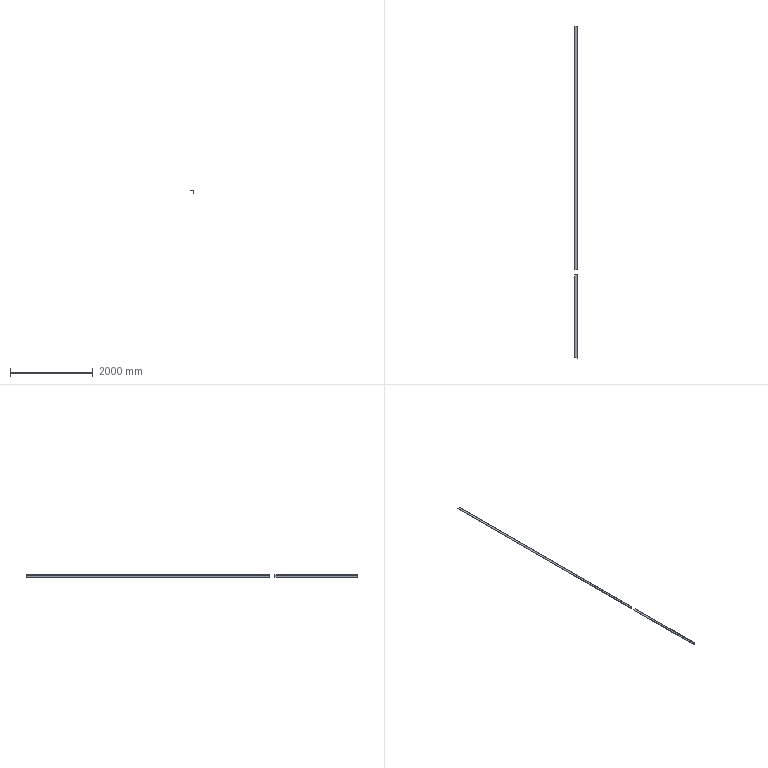Component | SolidWorks | 63#AngleIron-1 | 2 solids | 22 faces | box 63 x 8000 x 63 mm | volume 3919801 mm3 | plane 16 | cylinder 6 | commonest cylinder face diameters 2.667 x4 14 x2
STEP:
#1=CARTESIAN_POINT('',(81.493,-204.522,184.882));
#2=VERTEX_POINT('',#1);
#3=CARTESIAN_POINT('',(81.493,-283.262,184.882));
#4=VERTEX_POINT('',#3);
#5=CARTESIAN_POINT('',(81.493,31.699,184.882));
#6=DIRECTION('',(-0.,-1.,0.));
#7=VECTOR('',#6,39.37);
#8=LINE('',#5,#7);
#9=EDGE_CURVE('',#2,#4,#8,.T.);
#10=ORIENTED_EDGE('',*,*,#9,.F.);
#11=CARTESIAN_POINT('',(81.493,-204.522,187.362));
#12=VERTEX_POINT('',#11);
#13=CARTESIAN_POINT('',(81.493,-204.522,184.882));
#14=DIRECTION('',(0.,0.,1.));
#15=VECTOR('',#14,39.37);
#16=LINE('',#13,#15);
#17=EDGE_CURVE('',#2,#12,#16,.T.);
#18=ORIENTED_EDGE('',*,*,#17,.T.);
#19=CARTESIAN_POINT('',(81.493,-283.262,187.362));
#20=VERTEX_POINT('',#19);
#21=CARTESIAN_POINT('',(81.493,31.699,187.362));
#22=DIRECTION('',(-0.,-1.,0.));
#23=VECTOR('',#22,39.37);
#24=LINE('',#21,#23);
#25=EDGE_CURVE('',#12,#20,#24,.T.);
#26=ORIENTED_EDGE('',*,*,#25,.T.);
#27=CARTESIAN_POINT('',(81.493,-283.262,184.882));
#28=DIRECTION('',(-0.,-0.,-1.));
#29=VECTOR('',#28,39.37);
#30=LINE('',#27,#29);
#31=EDGE_CURVE('',#20,#4,#30,.T.);
#32=ORIENTED_EDGE('',*,*,#31,.T.);
#33=EDGE_LOOP('',(#10,#18,#26,#32));
#34=FACE_OUTER_BOUND('',#33,.T.);
#35=CARTESIAN_POINT('',(81.493,31.699,184.882));
#36=DIRECTION('',(-1.,0.,0.));
#37=DIRECTION('',(0.,1.,-0.));
#38=AXIS2_PLACEMENT_3D('',#35,#36,#37);
#39=PLANE('',#38);
#40=ADVANCED_FACE('',(#34),#39,.F.);
#41=CARTESIAN_POINT('',(81.388,-204.522,184.882));
#42=VERTEX_POINT('',#41);
#43=CARTESIAN_POINT('',(81.388,-283.262,184.882));
#44=VERTEX_POINT('',#43);
#45=CARTESIAN_POINT('',(81.388,31.699,184.882));
#46=DIRECTION('',(-0.,-1.,0.));
#47=VECTOR('',#46,39.37);
#48=LINE('',#45,#47);
#49=EDGE_CURVE('',#42,#44,#48,.T.);
#50=ORIENTED_EDGE('',*,*,#49,.F.);
#51=CARTESIAN_POINT('',(81.493,-204.522,184.882));
#52=DIRECTION('',(1.,0.,-0.));
#53=VECTOR('',#52,39.37);
#54=LINE('',#51,#53);
#55=EDGE_CURVE('',#42,#2,#54,.T.);
#56=ORIENTED_EDGE('',*,*,#55,.T.);
#57=ORIENTED_EDGE('',*,*,#9,.T.);
#58=CARTESIAN_POINT('',(81.493,-283.262,184.882));
#59=DIRECTION('',(-1.,0.,0.));
#60=VECTOR('',#59,39.37);
#61=LINE('',#58,#60);
#62=EDGE_CURVE('',#4,#44,#61,.T.);
#63=ORIENTED_EDGE('',*,*,#62,.T.);
#64=EDGE_LOOP('',(#50,#56,#57,#63));
#65=FACE_OUTER_BOUND('',#64,.T.);
#66=CARTESIAN_POINT('',(81.493,31.699,184.882));
#67=DIRECTION('',(0.,0.,1.));
#68=DIRECTION('',(1.,-0.,-0.));
#69=AXIS2_PLACEMENT_3D('',#66,#67,#68);
#70=PLANE('',#69);
#71=ADVANCED_FACE('',(#65),#70,.F.);
#72=CARTESIAN_POINT('',(81.336,-204.522,184.934));
#73=VERTEX_POINT('',#72);
#74=CARTESIAN_POINT('',(81.336,-283.262,184.934));
#75=VERTEX_POINT('',#74);
#76=CARTESIAN_POINT('',(81.336,31.699,184.934));
#77=DIRECTION('',(-0.,-1.,0.));
#78=VECTOR('',#77,39.37);
#79=LINE('',#76,#78);
#80=EDGE_CURVE('',#73,#75,#79,.T.);
#81=ORIENTED_EDGE('',*,*,#80,.F.);
#82=CARTESIAN_POINT('',(81.388,-204.522,184.934));
#83=DIRECTION('',(0.,-1.,-0.));
#84=DIRECTION('',(-1.,0.,0.));
#85=AXIS2_PLACEMENT_3D('',#82,#83,#84);
#86=CIRCLE('',#85,0.05249);
#87=EDGE_CURVE('',#73,#42,#86,.T.);
#88=ORIENTED_EDGE('',*,*,#87,.T.);
#89=ORIENTED_EDGE('',*,*,#49,.T.);
#90=CARTESIAN_POINT('',(81.388,-283.262,184.934));
#91=DIRECTION('',(0.,1.,-0.));
#92=DIRECTION('',(1.,0.,0.));
#93=AXIS2_PLACEMENT_3D('',#90,#91,#92);
#94=CIRCLE('',#93,0.05249);
#95=EDGE_CURVE('',#44,#75,#94,.T.);
#96=ORIENTED_EDGE('',*,*,#95,.T.);
#97=EDGE_LOOP('',(#81,#88,#89,#96));
#98=FACE_OUTER_BOUND('',#97,.T.);
#99=CARTESIAN_POINT('',(81.388,31.699,184.934));
#100=DIRECTION('',(-0.,-1.,0.));
#101=DIRECTION('',(-1.,0.,0.));
#102=AXIS2_PLACEMENT_3D('',#99,#100,#101);
#103=CYLINDRICAL_SURFACE('',#102,0.05249);
#104=ADVANCED_FACE('',(#98),#103,.T.);
#105=CARTESIAN_POINT('',(81.336,-204.522,186.929));
#106=VERTEX_POINT('',#105);
#107=CARTESIAN_POINT('',(81.336,-283.262,186.929));
#108=VERTEX_POINT('',#107);
#109=CARTESIAN_POINT('',(81.336,31.699,186.929));
#110=DIRECTION('',(-0.,-1.,0.));
#111=VECTOR('',#110,39.37);
#112=LINE('',#109,#111);
#113=EDGE_CURVE('',#106,#108,#112,.T.);
#114=ORIENTED_EDGE('',*,*,#113,.F.);
#115=CARTESIAN_POINT('',(81.336,-204.522,186.929));
#116=DIRECTION('',(-0.,-0.,-1.));
#117=VECTOR('',#116,39.37);
#118=LINE('',#115,#117);
#119=EDGE_CURVE('',#106,#73,#118,.T.);
#120=ORIENTED_EDGE('',*,*,#119,.T.);
#121=ORIENTED_EDGE('',*,*,#80,.T.);
#122=CARTESIAN_POINT('',(81.336,-283.262,186.929));
#123=DIRECTION('',(0.,0.,1.));
#124=VECTOR('',#123,39.37);
#125=LINE('',#122,#124);
#126=EDGE_CURVE('',#75,#108,#125,.T.);
#127=ORIENTED_EDGE('',*,*,#126,.T.);
#128=EDGE_LOOP('',(#114,#120,#121,#127));
#129=FACE_OUTER_BOUND('',#128,.T.);
#130=CARTESIAN_POINT('',(81.336,31.699,186.929));
#131=DIRECTION('',(1.,-0.,-0.));
#132=DIRECTION('',(-0.,-0.,-1.));
#133=AXIS2_PLACEMENT_3D('',#130,#131,#132);
#134=PLANE('',#133);
#135=ADVANCED_FACE('',(#129),#134,.F.);
#136=CARTESIAN_POINT('',(81.06,-204.522,187.205));
#137=VERTEX_POINT('',#136);
#138=CARTESIAN_POINT('',(81.06,-283.262,187.205));
#139=VERTEX_POINT('',#138);
#140=CARTESIAN_POINT('',(81.06,31.699,187.205));
#141=DIRECTION('',(-0.,-1.,0.));
#142=VECTOR('',#141,39.37);
#143=LINE('',#140,#142);
#144=EDGE_CURVE('',#137,#139,#143,.T.);
#145=ORIENTED_EDGE('',*,*,#144,.F.);
#146=CARTESIAN_POINT('',(81.06,-204.522,186.929));
#147=DIRECTION('',(0.,1.,0.));
#148=DIRECTION('',(-1.,0.,0.));
#149=AXIS2_PLACEMENT_3D('',#146,#147,#148);
#150=CIRCLE('',#149,0.2756);
#151=EDGE_CURVE('',#137,#106,#150,.T.);
#152=ORIENTED_EDGE('',*,*,#151,.T.);
#153=ORIENTED_EDGE('',*,*,#113,.T.);
#154=CARTESIAN_POINT('',(81.06,-283.262,186.929));
#155=DIRECTION('',(-0.,-1.,0.));
#156=DIRECTION('',(-1.,0.,0.));
#157=AXIS2_PLACEMENT_3D('',#154,#155,#156);
#158=CIRCLE('',#157,0.2756);
#159=EDGE_CURVE('',#108,#139,#158,.T.);
#160=ORIENTED_EDGE('',*,*,#159,.T.);
#161=EDGE_LOOP('',(#145,#152,#153,#160));
#162=FACE_OUTER_BOUND('',#161,.T.);
#163=CARTESIAN_POINT('',(81.06,31.699,186.929));
#164=DIRECTION('',(-0.,-1.,0.));
#165=DIRECTION('',(-1.,0.,0.));
#166=AXIS2_PLACEMENT_3D('',#163,#164,#165);
#167=CYLINDRICAL_SURFACE('',#166,0.2756);
#168=ADVANCED_FACE('',(#162),#167,.F.);
#169=CARTESIAN_POINT('',(79.065,-204.522,187.205));
#170=VERTEX_POINT('',#169);
#171=CARTESIAN_POINT('',(79.065,-283.262,187.205));
#172=VERTEX_POINT('',#171);
#173=CARTESIAN_POINT('',(79.065,31.699,187.205));
#174=DIRECTION('',(-0.,-1.,0.));
#175=VECTOR('',#174,39.37);
#176=LINE('',#173,#175);
#177=EDGE_CURVE('',#170,#172,#176,.T.);
#178=ORIENTED_EDGE('',*,*,#177,.F.);
#179=CARTESIAN_POINT('',(79.065,-204.522,187.205));
#180=DIRECTION('',(1.,0.,-0.));
#181=VECTOR('',#180,39.37);
#182=LINE('',#179,#181);
#183=EDGE_CURVE('',#170,#137,#182,.T.);
#184=ORIENTED_EDGE('',*,*,#183,.T.);
#185=ORIENTED_EDGE('',*,*,#144,.T.);
#186=CARTESIAN_POINT('',(79.065,-283.262,187.205));
#187=DIRECTION('',(-1.,0.,0.));
#188=VECTOR('',#187,39.37);
#189=LINE('',#186,#188);
#190=EDGE_CURVE('',#139,#172,#189,.T.);
#191=ORIENTED_EDGE('',*,*,#190,.T.);
#192=EDGE_LOOP('',(#178,#184,#185,#191));
#193=FACE_OUTER_BOUND('',#192,.T.);
#194=CARTESIAN_POINT('',(79.065,31.699,187.205));
#195=DIRECTION('',(0.,0.,1.));
#196=DIRECTION('',(1.,-0.,-0.));
#197=AXIS2_PLACEMENT_3D('',#194,#195,#196);
#198=PLANE('',#197);
#199=ADVANCED_FACE('',(#193),#198,.F.);
#200=CARTESIAN_POINT('',(79.013,-204.522,187.257));
#201=VERTEX_POINT('',#200);
#202=CARTESIAN_POINT('',(79.013,-283.262,187.257));
#203=VERTEX_POINT('',#202);
#204=CARTESIAN_POINT('',(79.013,31.699,187.257));
#205=DIRECTION('',(-0.,-1.,0.));
#206=VECTOR('',#205,39.37);
#207=LINE('',#204,#206);
#208=EDGE_CURVE('',#201,#203,#207,.T.);
#209=ORIENTED_EDGE('',*,*,#208,.F.);
#210=CARTESIAN_POINT('',(79.065,-204.522,187.257));
#211=DIRECTION('',(0.,-1.,-0.));
#212=DIRECTION('',(-1.,0.,0.));
#213=AXIS2_PLACEMENT_3D('',#210,#211,#212);
#214=CIRCLE('',#213,0.05249);
#215=EDGE_CURVE('',#201,#170,#214,.T.);
#216=ORIENTED_EDGE('',*,*,#215,.T.);
#217=ORIENTED_EDGE('',*,*,#177,.T.);
#218=CARTESIAN_POINT('',(79.065,-283.262,187.257));
#219=DIRECTION('',(0.,1.,-0.));
#220=DIRECTION('',(-1.,0.,0.));
#221=AXIS2_PLACEMENT_3D('',#218,#219,#220);
#222=CIRCLE('',#221,0.05249);
#223=EDGE_CURVE('',#172,#203,#222,.T.);
#224=ORIENTED_EDGE('',*,*,#223,.T.);
#225=EDGE_LOOP('',(#209,#216,#217,#224));
#226=FACE_OUTER_BOUND('',#225,.T.);
#227=CARTESIAN_POINT('',(79.065,31.699,187.257));
#228=DIRECTION('',(-0.,-1.,0.));
#229=DIRECTION('',(-1.,0.,0.));
#230=AXIS2_PLACEMENT_3D('',#227,#228,#229);
#231=CYLINDRICAL_SURFACE('',#230,0.05249);
#232=ADVANCED_FACE('',(#226),#231,.T.);
#233=CARTESIAN_POINT('',(79.013,-204.522,187.362));
#234=VERTEX_POINT('',#233);
#235=CARTESIAN_POINT('',(79.013,-283.262,187.362));
#236=VERTEX_POINT('',#235);
#237=CARTESIAN_POINT('',(79.013,31.699,187.362));
#238=DIRECTION('',(-0.,-1.,0.));
#239=VECTOR('',#238,39.37);
#240=LINE('',#237,#239);
#241=EDGE_CURVE('',#234,#236,#240,.T.);
#242=ORIENTED_EDGE('',*,*,#241,.F.);
#243=CARTESIAN_POINT('',(79.013,-204.522,187.362));
#244=DIRECTION('',(-0.,0.,-1.));
#245=VECTOR('',#244,39.37);
#246=LINE('',#243,#245);
#247=EDGE_CURVE('',#234,#201,#246,.T.);
#248=ORIENTED_EDGE('',*,*,#247,.T.);
#249=ORIENTED_EDGE('',*,*,#208,.T.);
#250=CARTESIAN_POINT('',(79.013,-283.262,187.362));
#251=DIRECTION('',(0.,0.,1.));
#252=VECTOR('',#251,39.37);
#253=LINE('',#250,#252);
#254=EDGE_CURVE('',#203,#236,#253,.T.);
#255=ORIENTED_EDGE('',*,*,#254,.T.);
#256=EDGE_LOOP('',(#242,#248,#249,#255));
#257=FACE_OUTER_BOUND('',#256,.T.);
#258=CARTESIAN_POINT('',(79.013,31.699,187.362));
#259=DIRECTION('',(1.,-0.,-0.));
#260=DIRECTION('',(-0.,-1.,0.));
#261=AXIS2_PLACEMENT_3D('',#258,#259,#260);
#262=PLANE('',#261);
#263=ADVANCED_FACE('',(#257),#262,.F.);
#264=ORIENTED_EDGE('',*,*,#25,.F.);
#265=CARTESIAN_POINT('',(81.493,-204.522,187.362));
#266=DIRECTION('',(-1.,0.,0.));
#267=VECTOR('',#266,39.37);
#268=LINE('',#265,#267);
#269=EDGE_CURVE('',#12,#234,#268,.T.);
#270=ORIENTED_EDGE('',*,*,#269,.T.);
#271=ORIENTED_EDGE('',*,*,#241,.T.);
#272=CARTESIAN_POINT('',(81.493,-283.262,187.362));
#273=DIRECTION('',(1.,-0.,-0.));
#274=VECTOR('',#273,39.37);
#275=LINE('',#272,#274);
#276=EDGE_CURVE('',#236,#20,#275,.T.);
#277=ORIENTED_EDGE('',*,*,#276,.T.);
#278=EDGE_LOOP('',(#264,#270,#271,#277));
#279=FACE_OUTER_BOUND('',#278,.T.);
#280=CARTESIAN_POINT('',(81.493,31.699,187.362));
#281=DIRECTION('',(-0.,-0.,-1.));
#282=DIRECTION('',(-1.,0.,0.));
#283=AXIS2_PLACEMENT_3D('',#280,#281,#282);
#284=PLANE('',#283);
#285=ADVANCED_FACE('',(#279),#284,.F.);
#286=ORIENTED_EDGE('',*,*,#31,.F.);
#287=ORIENTED_EDGE('',*,*,#276,.F.);
#288=ORIENTED_EDGE('',*,*,#254,.F.);
#289=ORIENTED_EDGE('',*,*,#223,.F.);
#290=ORIENTED_EDGE('',*,*,#190,.F.);
#291=ORIENTED_EDGE('',*,*,#159,.F.);
#292=ORIENTED_EDGE('',*,*,#126,.F.);
#293=ORIENTED_EDGE('',*,*,#95,.F.);
#294=ORIENTED_EDGE('',*,*,#62,.F.);
#295=EDGE_LOOP('',(#286,#287,#288,#289,#290,#291,#292,#293,#294));
#296=FACE_OUTER_BOUND('',#295,.T.);
#297=CARTESIAN_POINT('',(79.065,-283.262,187.257));
#298=DIRECTION('',(-0.,-1.,0.));
#299=DIRECTION('',(-1.,0.,0.));
#300=AXIS2_PLACEMENT_3D('',#297,#298,#299);
#301=PLANE('',#300);
#302=ADVANCED_FACE('',(#296),#301,.T.);
#303=ORIENTED_EDGE('',*,*,#55,.F.);
#304=ORIENTED_EDGE('',*,*,#87,.F.);
#305=ORIENTED_EDGE('',*,*,#119,.F.);
#306=ORIENTED_EDGE('',*,*,#151,.F.);
#307=ORIENTED_EDGE('',*,*,#183,.F.);
#308=ORIENTED_EDGE('',*,*,#215,.F.);
#309=ORIENTED_EDGE('',*,*,#247,.F.);
#310=ORIENTED_EDGE('',*,*,#269,.F.);
#311=ORIENTED_EDGE('',*,*,#17,.F.);
#312=EDGE_LOOP('',(#303,#304,#305,#306,#307,#308,#309,#310,#311));
#313=FACE_OUTER_BOUND('',#312,.T.);
#314=CARTESIAN_POINT('',(-68.113,-204.522,23.622));
#315=DIRECTION('',(0.,-1.,0.));
#316=DIRECTION('',(0.,-0.,-1.));
#317=AXIS2_PLACEMENT_3D('',#314,#315,#316);
#318=PLANE('',#317);
#319=ADVANCED_FACE('',(#313),#318,.F.);
#320=CLOSED_SHELL('',(#40,#71,#104,#135,#168,#199,#232,#263,#285,#302,#319));
#321=MANIFOLD_SOLID_BREP('',#320);
#322=CARTESIAN_POINT('',(81.493,31.699,187.362));
#323=VERTEX_POINT('',#322);
#324=CARTESIAN_POINT('',(81.493,31.699,184.882));
#325=VERTEX_POINT('',#324);
#326=CARTESIAN_POINT('',(81.493,31.699,184.882));
#327=DIRECTION('',(-0.,-0.,-1.));
#328=VECTOR('',#327,39.37);
#329=LINE('',#326,#328);
#330=EDGE_CURVE('',#323,#325,#329,.T.);
#331=ORIENTED_EDGE('',*,*,#330,.T.);
#332=CARTESIAN_POINT('',(81.388,31.699,184.882));
#333=VERTEX_POINT('',#332);
#334=CARTESIAN_POINT('',(81.493,31.699,184.882));
#335=DIRECTION('',(-1.,0.,0.));
#336=VECTOR('',#335,39.37);
#337=LINE('',#334,#336);
#338=EDGE_CURVE('',#325,#333,#337,.T.);
#339=ORIENTED_EDGE('',*,*,#338,.T.);
#340=CARTESIAN_POINT('',(81.336,31.699,184.934));
#341=VERTEX_POINT('',#340);
#342=CARTESIAN_POINT('',(81.388,31.699,184.934));
#343=DIRECTION('',(0.,1.,-0.));
#344=DIRECTION('',(1.,0.,0.));
#345=AXIS2_PLACEMENT_3D('',#342,#343,#344);
#346=CIRCLE('',#345,0.05249);
#347=EDGE_CURVE('',#333,#341,#346,.T.);
#348=ORIENTED_EDGE('',*,*,#347,.T.);
#349=CARTESIAN_POINT('',(81.336,31.699,186.929));
#350=VERTEX_POINT('',#349);
#351=CARTESIAN_POINT('',(81.336,31.699,186.929));
#352=DIRECTION('',(0.,0.,1.));
#353=VECTOR('',#352,39.37);
#354=LINE('',#351,#353);
#355=EDGE_CURVE('',#341,#350,#354,.T.);
#356=ORIENTED_EDGE('',*,*,#355,.T.);
#357=CARTESIAN_POINT('',(81.06,31.699,187.205));
#358=VERTEX_POINT('',#357);
#359=CARTESIAN_POINT('',(81.06,31.699,186.929));
#360=DIRECTION('',(-0.,-1.,0.));
#361=DIRECTION('',(-1.,0.,0.));
#362=AXIS2_PLACEMENT_3D('',#359,#360,#361);
#363=CIRCLE('',#362,0.2756);
#364=EDGE_CURVE('',#350,#358,#363,.T.);
#365=ORIENTED_EDGE('',*,*,#364,.T.);
#366=CARTESIAN_POINT('',(79.065,31.699,187.205));
#367=VERTEX_POINT('',#366);
#368=CARTESIAN_POINT('',(79.065,31.699,187.205));
#369=DIRECTION('',(-1.,0.,0.));
#370=VECTOR('',#369,39.37);
#371=LINE('',#368,#370);
#372=EDGE_CURVE('',#358,#367,#371,.T.);
#373=ORIENTED_EDGE('',*,*,#372,.T.);
#374=CARTESIAN_POINT('',(79.013,31.699,187.257));
#375=VERTEX_POINT('',#374);
#376=CARTESIAN_POINT('',(79.065,31.699,187.257));
#377=DIRECTION('',(0.,1.,-0.));
#378=DIRECTION('',(-1.,0.,0.));
#379=AXIS2_PLACEMENT_3D('',#376,#377,#378);
#380=CIRCLE('',#379,0.05249);
#381=EDGE_CURVE('',#367,#375,#380,.T.);
#382=ORIENTED_EDGE('',*,*,#381,.T.);
#383=CARTESIAN_POINT('',(79.013,31.699,187.362));
#384=VERTEX_POINT('',#383);
#385=CARTESIAN_POINT('',(79.013,31.699,187.362));
#386=DIRECTION('',(0.,0.,1.));
#387=VECTOR('',#386,39.37);
#388=LINE('',#385,#387);
#389=EDGE_CURVE('',#375,#384,#388,.T.);
#390=ORIENTED_EDGE('',*,*,#389,.T.);
#391=CARTESIAN_POINT('',(81.493,31.699,187.362));
#392=DIRECTION('',(1.,-0.,-0.));
#393=VECTOR('',#392,39.37);
#394=LINE('',#391,#393);
#395=EDGE_CURVE('',#384,#323,#394,.T.);
#396=ORIENTED_EDGE('',*,*,#395,.T.);
#397=EDGE_LOOP('',(#331,#339,#348,#356,#365,#373,#382,#390,#396));
#398=FACE_OUTER_BOUND('',#397,.T.);
#399=CARTESIAN_POINT('',(79.065,31.699,187.257));
#400=DIRECTION('',(-0.,-1.,0.));
#401=DIRECTION('',(-1.,0.,0.));
#402=AXIS2_PLACEMENT_3D('',#399,#400,#401);
#403=PLANE('',#402);
#404=ADVANCED_FACE('',(#398),#403,.F.);
#405=CARTESIAN_POINT('',(79.013,-199.6,187.362));
#406=VERTEX_POINT('',#405);
#407=CARTESIAN_POINT('',(79.013,31.699,187.362));
#408=DIRECTION('',(-0.,-1.,0.));
#409=VECTOR('',#408,39.37);
#410=LINE('',#407,#409);
#411=EDGE_CURVE('',#384,#406,#410,.T.);
#412=ORIENTED_EDGE('',*,*,#411,.T.);
#413=CARTESIAN_POINT('',(81.493,-199.6,187.362));
#414=VERTEX_POINT('',#413);
#415=CARTESIAN_POINT('',(81.493,-199.6,187.362));
#416=DIRECTION('',(1.,0.,-0.));
#417=VECTOR('',#416,39.37);
#418=LINE('',#415,#417);
#419=EDGE_CURVE('',#406,#414,#418,.T.);
#420=ORIENTED_EDGE('',*,*,#419,.T.);
#421=CARTESIAN_POINT('',(81.493,31.699,187.362));
#422=DIRECTION('',(-0.,-1.,0.));
#423=VECTOR('',#422,39.37);
#424=LINE('',#421,#423);
#425=EDGE_CURVE('',#323,#414,#424,.T.);
#426=ORIENTED_EDGE('',*,*,#425,.F.);
#427=ORIENTED_EDGE('',*,*,#395,.F.);
#428=EDGE_LOOP('',(#412,#420,#426,#427));
#429=FACE_OUTER_BOUND('',#428,.T.);
#430=CARTESIAN_POINT('',(81.493,31.699,187.362));
#431=DIRECTION('',(-0.,-0.,-1.));
#432=DIRECTION('',(-1.,0.,0.));
#433=AXIS2_PLACEMENT_3D('',#430,#431,#432);
#434=PLANE('',#433);
#435=ADVANCED_FACE('',(#429),#434,.F.);
#436=CARTESIAN_POINT('',(79.013,-199.6,187.257));
#437=VERTEX_POINT('',#436);
#438=CARTESIAN_POINT('',(79.013,31.699,187.257));
#439=DIRECTION('',(-0.,-1.,0.));
#440=VECTOR('',#439,39.37);
#441=LINE('',#438,#440);
#442=EDGE_CURVE('',#375,#437,#441,.T.);
#443=ORIENTED_EDGE('',*,*,#442,.T.);
#444=CARTESIAN_POINT('',(79.013,-199.6,187.362));
#445=DIRECTION('',(0.,0.,1.));
#446=VECTOR('',#445,39.37);
#447=LINE('',#444,#446);
#448=EDGE_CURVE('',#437,#406,#447,.T.);
#449=ORIENTED_EDGE('',*,*,#448,.T.);
#450=ORIENTED_EDGE('',*,*,#411,.F.);
#451=ORIENTED_EDGE('',*,*,#389,.F.);
#452=EDGE_LOOP('',(#443,#449,#450,#451));
#453=FACE_OUTER_BOUND('',#452,.T.);
#454=CARTESIAN_POINT('',(79.013,31.699,187.362));
#455=DIRECTION('',(1.,-0.,-0.));
#456=DIRECTION('',(-0.,-1.,0.));
#457=AXIS2_PLACEMENT_3D('',#454,#455,#456);
#458=PLANE('',#457);
#459=ADVANCED_FACE('',(#453),#458,.F.);
#460=CARTESIAN_POINT('',(79.065,-199.6,187.205));
#461=VERTEX_POINT('',#460);
#462=CARTESIAN_POINT('',(79.065,31.699,187.205));
#463=DIRECTION('',(-0.,-1.,0.));
#464=VECTOR('',#463,39.37);
#465=LINE('',#462,#464);
#466=EDGE_CURVE('',#367,#461,#465,.T.);
#467=ORIENTED_EDGE('',*,*,#466,.T.);
#468=CARTESIAN_POINT('',(79.065,-199.6,187.257));
#469=DIRECTION('',(0.,1.,0.));
#470=DIRECTION('',(1.,0.,0.));
#471=AXIS2_PLACEMENT_3D('',#468,#469,#470);
#472=CIRCLE('',#471,0.05249);
#473=EDGE_CURVE('',#461,#437,#472,.T.);
#474=ORIENTED_EDGE('',*,*,#473,.T.);
#475=ORIENTED_EDGE('',*,*,#442,.F.);
#476=ORIENTED_EDGE('',*,*,#381,.F.);
#477=EDGE_LOOP('',(#467,#474,#475,#476));
#478=FACE_OUTER_BOUND('',#477,.T.);
#479=CARTESIAN_POINT('',(79.065,31.699,187.257));
#480=DIRECTION('',(-0.,-1.,0.));
#481=DIRECTION('',(-1.,0.,0.));
#482=AXIS2_PLACEMENT_3D('',#479,#480,#481);
#483=CYLINDRICAL_SURFACE('',#482,0.05249);
#484=ADVANCED_FACE('',(#478),#483,.T.);
#485=CARTESIAN_POINT('',(81.06,-199.6,187.205));
#486=VERTEX_POINT('',#485);
#487=CARTESIAN_POINT('',(81.06,31.699,187.205));
#488=DIRECTION('',(-0.,-1.,0.));
#489=VECTOR('',#488,39.37);
#490=LINE('',#487,#489);
#491=EDGE_CURVE('',#358,#486,#490,.T.);
#492=ORIENTED_EDGE('',*,*,#491,.T.);
#493=CARTESIAN_POINT('',(79.065,-199.6,187.205));
#494=DIRECTION('',(-1.,0.,0.));
#495=VECTOR('',#494,39.37);
#496=LINE('',#493,#495);
#497=EDGE_CURVE('',#486,#461,#496,.T.);
#498=ORIENTED_EDGE('',*,*,#497,.T.);
#499=ORIENTED_EDGE('',*,*,#466,.F.);
#500=ORIENTED_EDGE('',*,*,#372,.F.);
#501=EDGE_LOOP('',(#492,#498,#499,#500));
#502=FACE_OUTER_BOUND('',#501,.T.);
#503=CARTESIAN_POINT('',(79.065,31.699,187.205));
#504=DIRECTION('',(0.,0.,1.));
#505=DIRECTION('',(1.,-0.,-0.));
#506=AXIS2_PLACEMENT_3D('',#503,#504,#505);
#507=PLANE('',#506);
#508=ADVANCED_FACE('',(#502),#507,.F.);
#509=CARTESIAN_POINT('',(81.336,-199.6,186.929));
#510=VERTEX_POINT('',#509);
#511=CARTESIAN_POINT('',(81.336,31.699,186.929));
#512=DIRECTION('',(-0.,-1.,0.));
#513=VECTOR('',#512,39.37);
#514=LINE('',#511,#513);
#515=EDGE_CURVE('',#350,#510,#514,.T.);
#516=ORIENTED_EDGE('',*,*,#515,.T.);
#517=CARTESIAN_POINT('',(81.06,-199.6,186.929));
#518=DIRECTION('',(0.,-1.,-0.));
#519=DIRECTION('',(1.,0.,0.));
#520=AXIS2_PLACEMENT_3D('',#517,#518,#519);
#521=CIRCLE('',#520,0.2756);
#522=EDGE_CURVE('',#510,#486,#521,.T.);
#523=ORIENTED_EDGE('',*,*,#522,.T.);
#524=ORIENTED_EDGE('',*,*,#491,.F.);
#525=ORIENTED_EDGE('',*,*,#364,.F.);
#526=EDGE_LOOP('',(#516,#523,#524,#525));
#527=FACE_OUTER_BOUND('',#526,.T.);
#528=CARTESIAN_POINT('',(81.06,31.699,186.929));
#529=DIRECTION('',(-0.,-1.,0.));
#530=DIRECTION('',(-1.,0.,0.));
#531=AXIS2_PLACEMENT_3D('',#528,#529,#530);
#532=CYLINDRICAL_SURFACE('',#531,0.2756);
#533=ADVANCED_FACE('',(#527),#532,.F.);
#534=CARTESIAN_POINT('',(81.336,-199.6,184.934));
#535=VERTEX_POINT('',#534);
#536=CARTESIAN_POINT('',(81.336,31.699,184.934));
#537=DIRECTION('',(-0.,-1.,0.));
#538=VECTOR('',#537,39.37);
#539=LINE('',#536,#538);
#540=EDGE_CURVE('',#341,#535,#539,.T.);
#541=ORIENTED_EDGE('',*,*,#540,.T.);
#542=CARTESIAN_POINT('',(81.336,-199.6,186.929));
#543=DIRECTION('',(0.,0.,1.));
#544=VECTOR('',#543,39.37);
#545=LINE('',#542,#544);
#546=EDGE_CURVE('',#535,#510,#545,.T.);
#547=ORIENTED_EDGE('',*,*,#546,.T.);
#548=ORIENTED_EDGE('',*,*,#515,.F.);
#549=ORIENTED_EDGE('',*,*,#355,.F.);
#550=EDGE_LOOP('',(#541,#547,#548,#549));
#551=FACE_OUTER_BOUND('',#550,.T.);
#552=CARTESIAN_POINT('',(81.336,31.699,186.929));
#553=DIRECTION('',(1.,-0.,-0.));
#554=DIRECTION('',(-0.,-0.,-1.));
#555=AXIS2_PLACEMENT_3D('',#552,#553,#554);
#556=PLANE('',#555);
#557=ADVANCED_FACE('',(#551),#556,.F.);
#558=CARTESIAN_POINT('',(81.388,-199.6,184.882));
#559=VERTEX_POINT('',#558);
#560=CARTESIAN_POINT('',(81.388,31.699,184.882));
#561=DIRECTION('',(-0.,-1.,0.));
#562=VECTOR('',#561,39.37);
#563=LINE('',#560,#562);
#564=EDGE_CURVE('',#333,#559,#563,.T.);
#565=ORIENTED_EDGE('',*,*,#564,.T.);
#566=CARTESIAN_POINT('',(81.388,-199.6,184.934));
#567=DIRECTION('',(0.,1.,0.));
#568=DIRECTION('',(1.,0.,0.));
#569=AXIS2_PLACEMENT_3D('',#566,#567,#568);
#570=CIRCLE('',#569,0.05249);
#571=EDGE_CURVE('',#559,#535,#570,.T.);
#572=ORIENTED_EDGE('',*,*,#571,.T.);
#573=ORIENTED_EDGE('',*,*,#540,.F.);
#574=ORIENTED_EDGE('',*,*,#347,.F.);
#575=EDGE_LOOP('',(#565,#572,#573,#574));
#576=FACE_OUTER_BOUND('',#575,.T.);
#577=CARTESIAN_POINT('',(81.388,31.699,184.934));
#578=DIRECTION('',(-0.,-1.,0.));
#579=DIRECTION('',(-1.,0.,0.));
#580=AXIS2_PLACEMENT_3D('',#577,#578,#579);
#581=CYLINDRICAL_SURFACE('',#580,0.05249);
#582=ADVANCED_FACE('',(#576),#581,.T.);
#583=CARTESIAN_POINT('',(81.493,-199.6,184.882));
#584=VERTEX_POINT('',#583);
#585=CARTESIAN_POINT('',(81.493,31.699,184.882));
#586=DIRECTION('',(-0.,-1.,0.));
#587=VECTOR('',#586,39.37);
#588=LINE('',#585,#587);
#589=EDGE_CURVE('',#325,#584,#588,.T.);
#590=ORIENTED_EDGE('',*,*,#589,.T.);
#591=CARTESIAN_POINT('',(81.493,-199.6,184.882));
#592=DIRECTION('',(-1.,0.,0.));
#593=VECTOR('',#592,39.37);
#594=LINE('',#591,#593);
#595=EDGE_CURVE('',#584,#559,#594,.T.);
#596=ORIENTED_EDGE('',*,*,#595,.T.);
#597=ORIENTED_EDGE('',*,*,#564,.F.);
#598=ORIENTED_EDGE('',*,*,#338,.F.);
#599=EDGE_LOOP('',(#590,#596,#597,#598));
#600=FACE_OUTER_BOUND('',#599,.T.);
#601=CARTESIAN_POINT('',(81.493,31.699,184.882));
#602=DIRECTION('',(0.,0.,1.));
#603=DIRECTION('',(1.,-0.,-0.));
#604=AXIS2_PLACEMENT_3D('',#601,#602,#603);
#605=PLANE('',#604);
#606=ADVANCED_FACE('',(#600),#605,.F.);
#607=ORIENTED_EDGE('',*,*,#425,.T.);
#608=CARTESIAN_POINT('',(81.493,-199.6,184.882));
#609=DIRECTION('',(-0.,0.,-1.));
#610=VECTOR('',#609,39.37);
#611=LINE('',#608,#610);
#612=EDGE_CURVE('',#414,#584,#611,.T.);
#613=ORIENTED_EDGE('',*,*,#612,.T.);
#614=ORIENTED_EDGE('',*,*,#589,.F.);
#615=ORIENTED_EDGE('',*,*,#330,.F.);
#616=EDGE_LOOP('',(#607,#613,#614,#615));
#617=FACE_OUTER_BOUND('',#616,.T.);
#618=CARTESIAN_POINT('',(81.493,31.699,184.882));
#619=DIRECTION('',(-1.,0.,0.));
#620=DIRECTION('',(0.,1.,-0.));
#621=AXIS2_PLACEMENT_3D('',#618,#619,#620);
#622=PLANE('',#621);
#623=ADVANCED_FACE('',(#617),#622,.F.);
#624=ORIENTED_EDGE('',*,*,#419,.F.);
#625=ORIENTED_EDGE('',*,*,#448,.F.);
#626=ORIENTED_EDGE('',*,*,#473,.F.);
#627=ORIENTED_EDGE('',*,*,#497,.F.);
#628=ORIENTED_EDGE('',*,*,#522,.F.);
#629=ORIENTED_EDGE('',*,*,#546,.F.);
#630=ORIENTED_EDGE('',*,*,#571,.F.);
#631=ORIENTED_EDGE('',*,*,#595,.F.);
#632=ORIENTED_EDGE('',*,*,#612,.F.);
#633=EDGE_LOOP('',(#624,#625,#626,#627,#628,#629,#630,#631,#632));
#634=FACE_OUTER_BOUND('',#633,.T.);
#635=CARTESIAN_POINT('',(-68.113,-199.6,23.622));
#636=DIRECTION('',(0.,1.,-0.));
#637=DIRECTION('',(0.,0.,1.));
#638=AXIS2_PLACEMENT_3D('',#635,#636,#637);
#639=PLANE('',#638);
#640=ADVANCED_FACE('',(#634),#639,.F.);
#641=CLOSED_SHELL('',(#404,#435,#459,#484,#508,#533,#557,#582,#606,#623,#640));
#642=MANIFOLD_SOLID_BREP('',#641);
#643=CARTESIAN_POINT('',(0.,0.,0.));
#644=DIRECTION('',(0.,0.,1.));
#645=DIRECTION('',(1.,0.,0.));
#646=AXIS2_PLACEMENT_3D('',#643,#644,#645);
#647=(LENGTH_UNIT()NAMED_UNIT(*)SI_UNIT($,.METRE.));
#648=LENGTH_MEASURE_WITH_UNIT(LENGTH_MEASURE(0.0254),#647);
#649=DIMENSIONAL_EXPONENTS(1.,0.,0.,0.,0.,0.,0.);
#650=(CONVERSION_BASED_UNIT('',#648)LENGTH_UNIT()NAMED_UNIT(#649));
#651=UNCERTAINTY_MEASURE_WITH_UNIT(LENGTH_MEASURE(0.00001),#650,'','');
#652=(NAMED_UNIT(*)PLANE_ANGLE_UNIT()SI_UNIT($,.RADIAN.));
#653=(NAMED_UNIT(*)SI_UNIT($,.STERADIAN.)SOLID_ANGLE_UNIT());
#654=(GEOMETRIC_REPRESENTATION_CONTEXT(3)GLOBAL_UNCERTAINTY_ASSIGNED_CONTEXT((#651))GLOBAL_UNIT_ASSIGNED_CONTEXT((#650,#652,#653))REPRESENTATION_CONTEXT('',''));
#655=ADVANCED_BREP_SHAPE_REPRESENTATION('',(#321,#642,#646),#654);
#656=COLOUR_RGB('',0.7922,0.8196,0.9333);
#657=FILL_AREA_STYLE_COLOUR('',#656);
#658=FILL_AREA_STYLE('',(#657));
#659=SURFACE_STYLE_FILL_AREA(#658);
#660=SURFACE_SIDE_STYLE('',(#659));
#661=SURFACE_STYLE_USAGE(.BOTH.,#660);
#662=PRESENTATION_STYLE_ASSIGNMENT((#661));
#663=STYLED_ITEM('',(#662),#321);
#664=PRESENTATION_LAYER_ASSIGNMENT('','',(#663));
#665=COLOUR_RGB('',0.7922,0.8196,0.9333);
#666=FILL_AREA_STYLE_COLOUR('',#665);
#667=FILL_AREA_STYLE('',(#666));
#668=SURFACE_STYLE_FILL_AREA(#667);
#669=SURFACE_SIDE_STYLE('',(#668));
#670=SURFACE_STYLE_USAGE(.BOTH.,#669);
#671=PRESENTATION_STYLE_ASSIGNMENT((#670));
#672=STYLED_ITEM('',(#671),#642);
#673=PRESENTATION_LAYER_ASSIGNMENT('','',(#672));
#674=(LENGTH_UNIT()NAMED_UNIT(*)SI_UNIT($,.METRE.));
#675=LENGTH_MEASURE_WITH_UNIT(LENGTH_MEASURE(0.0254),#674);
#676=DIMENSIONAL_EXPONENTS(1.,0.,0.,0.,0.,0.,0.);
#677=(CONVERSION_BASED_UNIT('',#675)LENGTH_UNIT()NAMED_UNIT(#676));
#678=UNCERTAINTY_MEASURE_WITH_UNIT(LENGTH_MEASURE(0.00001),#677,'','');
#679=(NAMED_UNIT(*)PLANE_ANGLE_UNIT()SI_UNIT($,.RADIAN.));
#680=(NAMED_UNIT(*)SI_UNIT($,.STERADIAN.)SOLID_ANGLE_UNIT());
#681=(GEOMETRIC_REPRESENTATION_CONTEXT(3)GLOBAL_UNCERTAINTY_ASSIGNED_CONTEXT((#678))GLOBAL_UNIT_ASSIGNED_CONTEXT((#677,#679,#680))REPRESENTATION_CONTEXT('',''));
#682=MECHANICAL_DESIGN_GEOMETRIC_PRESENTATION_REPRESENTATION('',(#672),#681);
#683=(LENGTH_UNIT()NAMED_UNIT(*)SI_UNIT($,.METRE.));
#684=LENGTH_MEASURE_WITH_UNIT(LENGTH_MEASURE(0.0254),#683);
#685=DIMENSIONAL_EXPONENTS(1.,0.,0.,0.,0.,0.,0.);
#686=(CONVERSION_BASED_UNIT('',#684)LENGTH_UNIT()NAMED_UNIT(#685));
#687=UNCERTAINTY_MEASURE_WITH_UNIT(LENGTH_MEASURE(0.00001),#686,'','');
#688=(NAMED_UNIT(*)PLANE_ANGLE_UNIT()SI_UNIT($,.RADIAN.));
#689=(NAMED_UNIT(*)SI_UNIT($,.STERADIAN.)SOLID_ANGLE_UNIT());
#690=(GEOMETRIC_REPRESENTATION_CONTEXT(3)GLOBAL_UNCERTAINTY_ASSIGNED_CONTEXT((#687))GLOBAL_UNIT_ASSIGNED_CONTEXT((#686,#688,#689))REPRESENTATION_CONTEXT('',''));
#691=MECHANICAL_DESIGN_GEOMETRIC_PRESENTATION_REPRESENTATION('',(#663),#690);